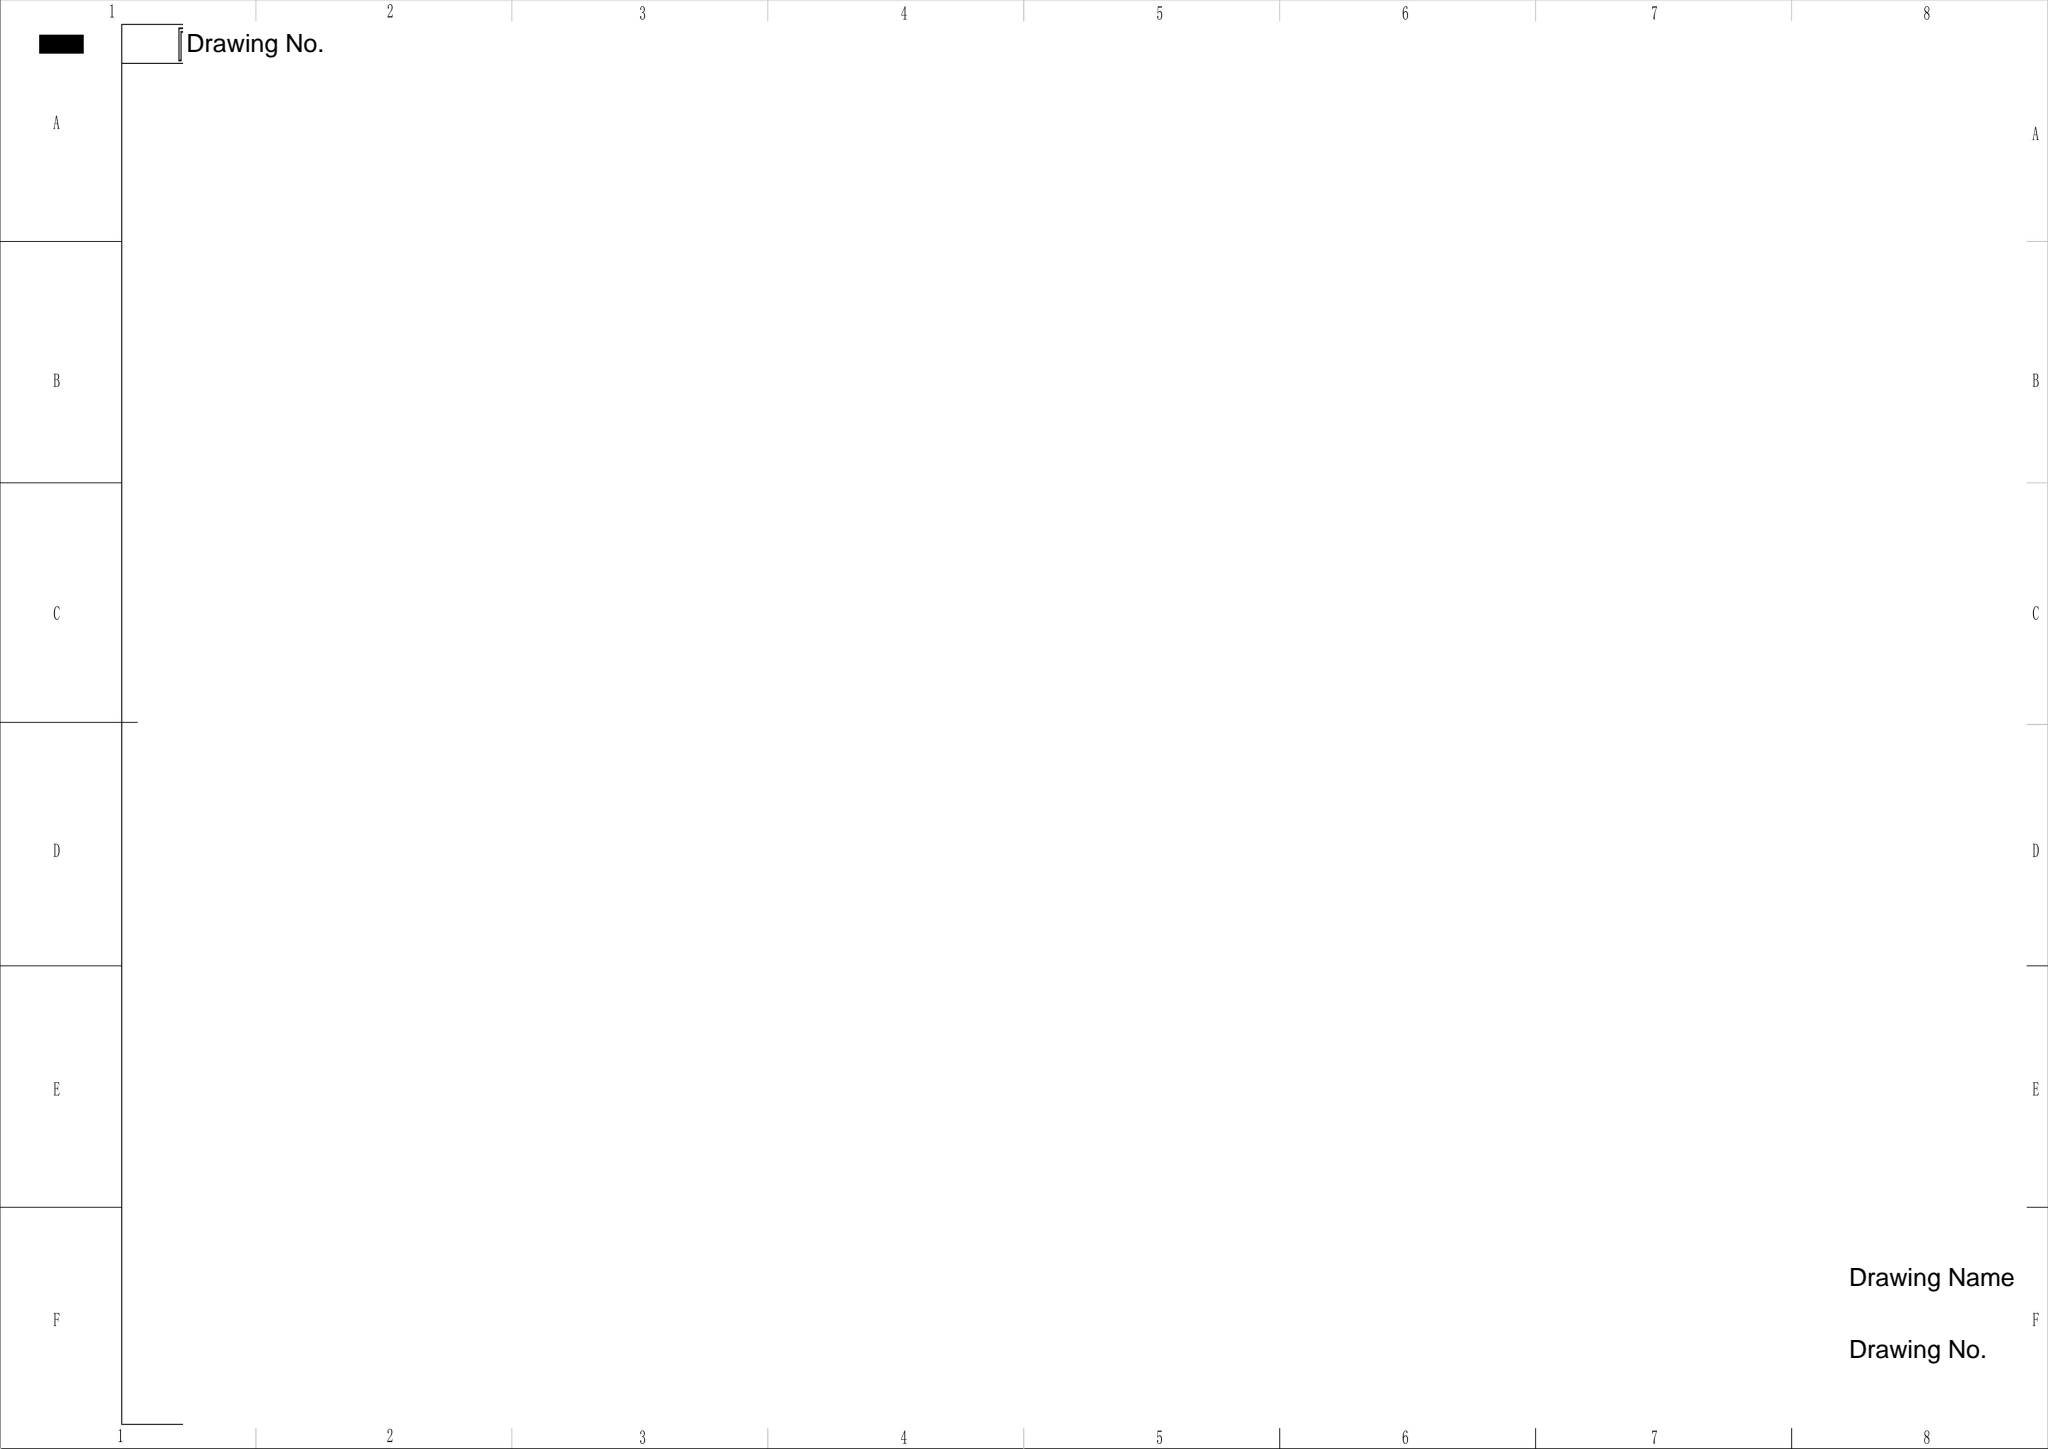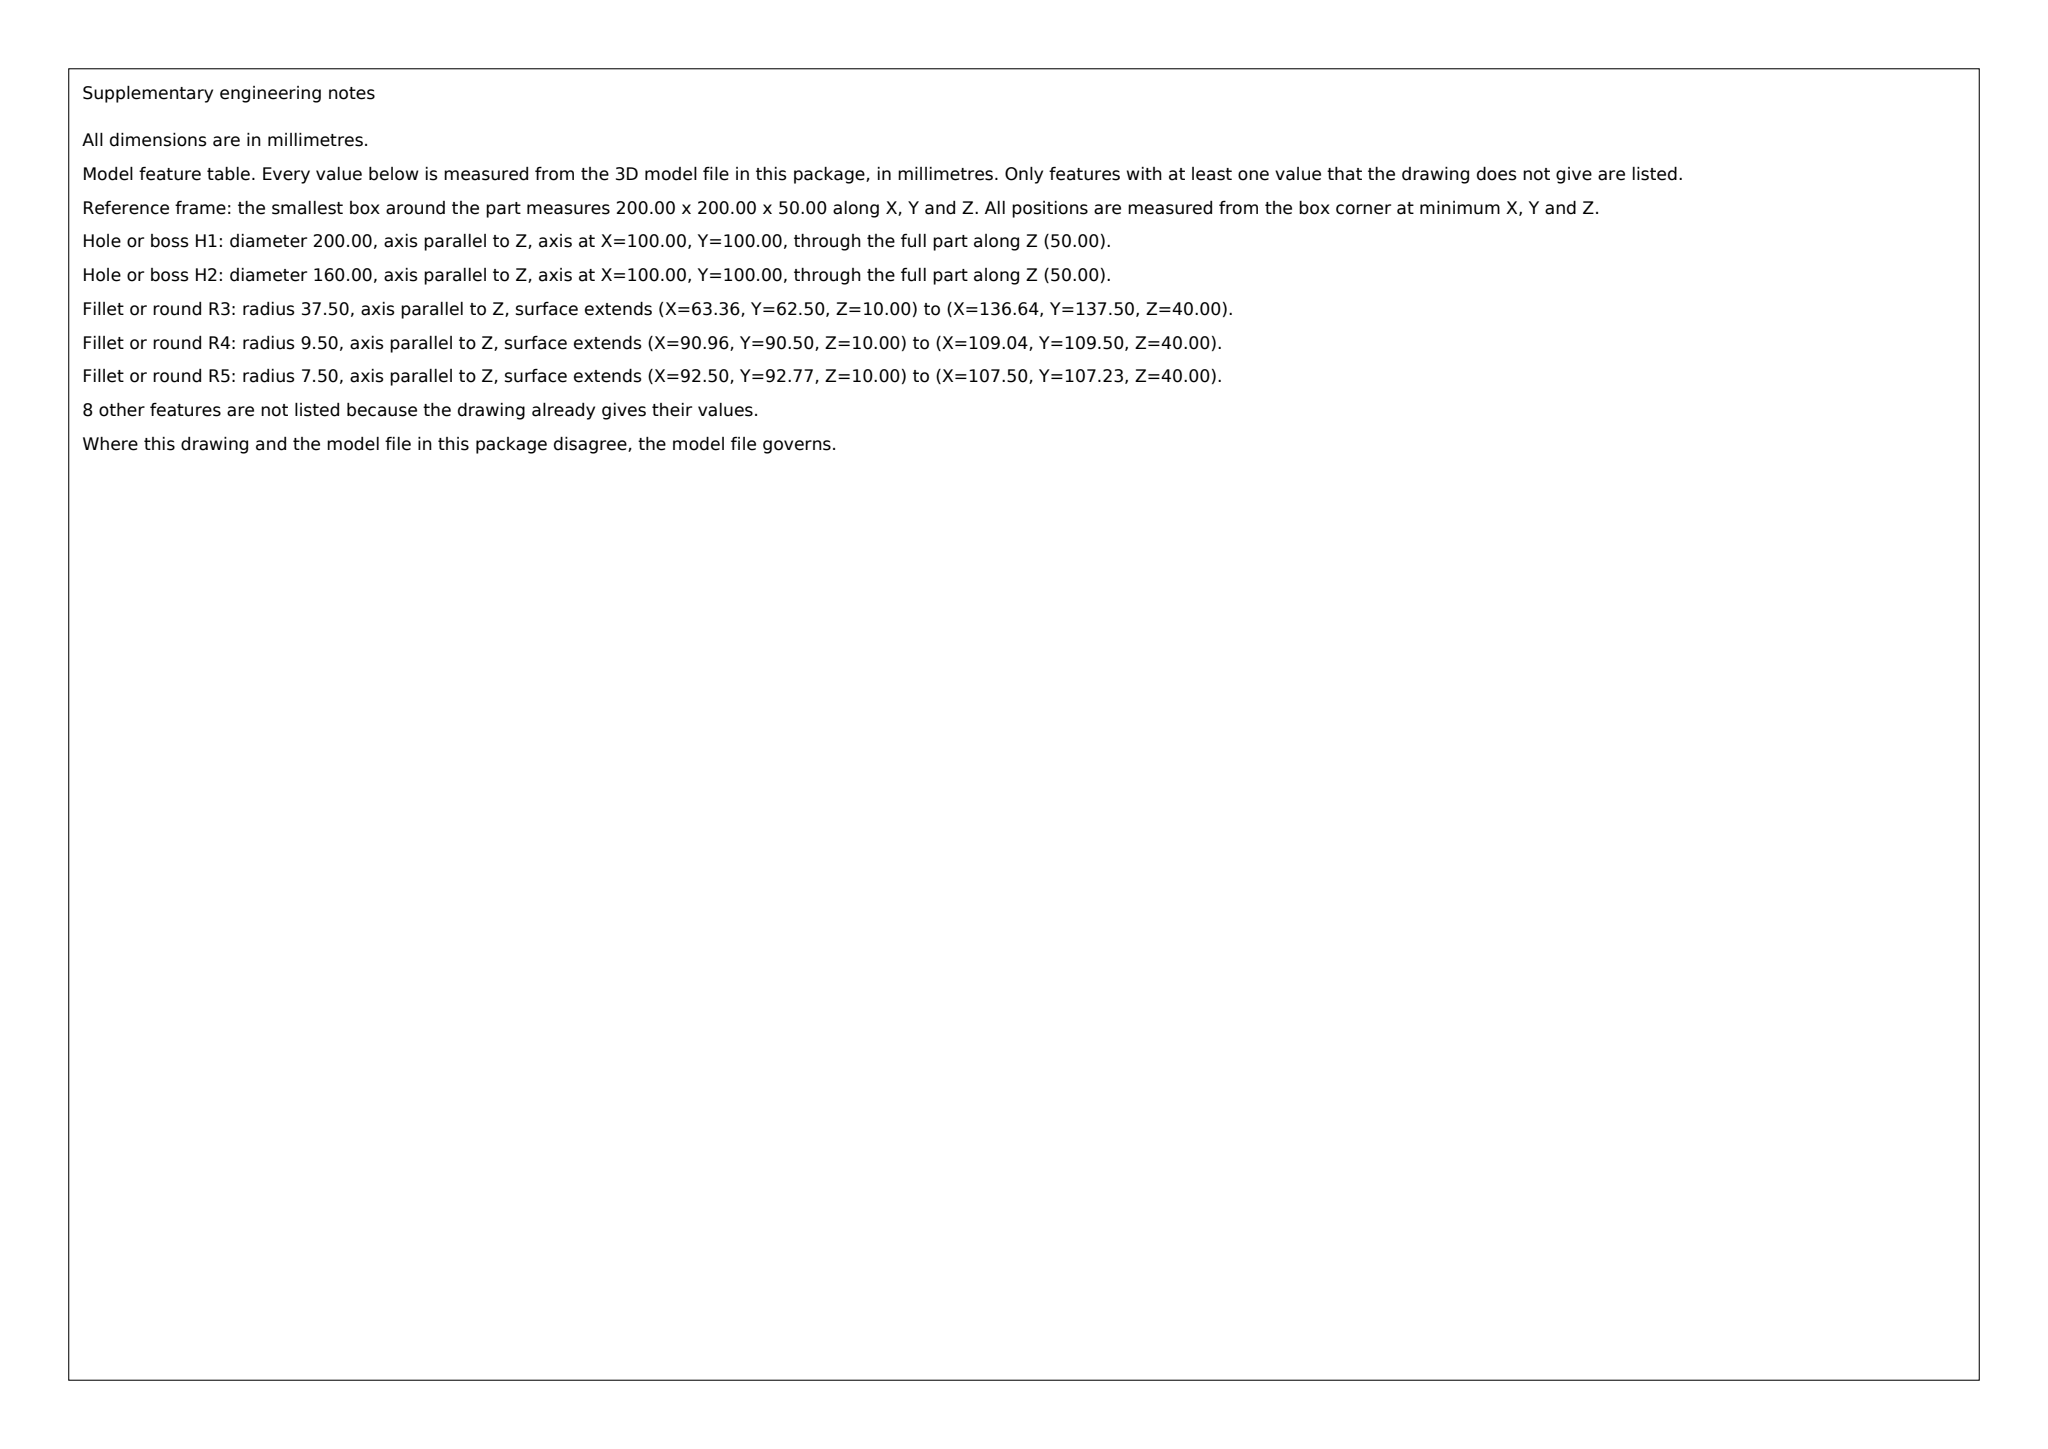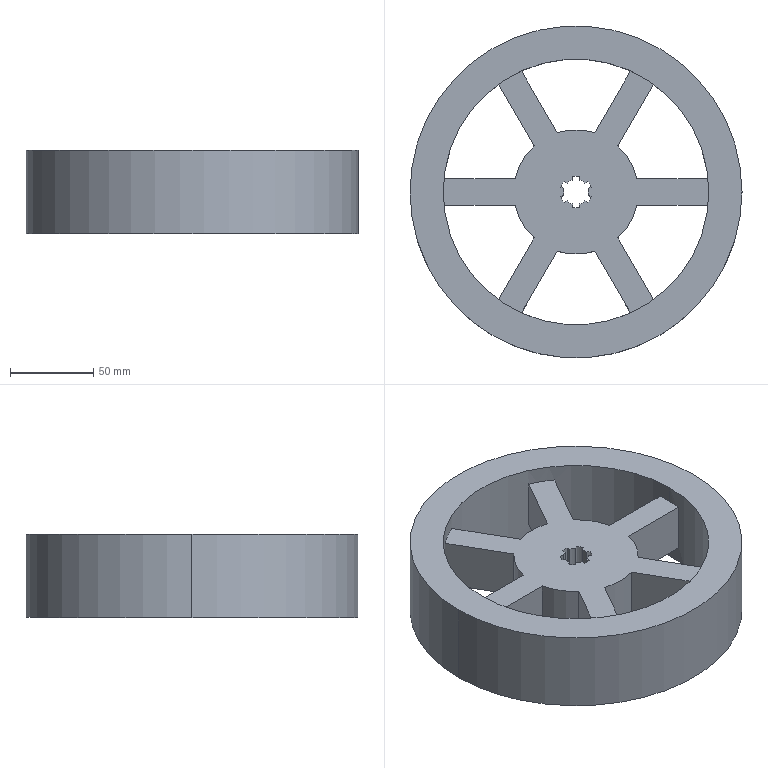Part | SolidWorks | mm | 1 solid | 51 faces | box 200 x 200 x 50 mm | volume 814108 mm3 | plane 28 | cylinder 23 | commonest cylinder face diameters 15 x7 75 x6 19 x6 160 x2 200 x2
build123d program:
from build123d import *

# Parameters (mm, degrees)
SKETCH1_R           = 100
BOSS_EXTRUDE1_DEPTH = 25
SKETCH2_R           = 80
CUT_EXTRUDE1_DEPTH  = 10
CUT_EXTRUDE3_DEPTH  = 147.969
CUT_EXTRUDE4_DEPTH  = 147.969


with BuildPart() as part:
    # Sketch1 → Boss-Extrude1 (new, symmetric)
    with BuildSketch(Plane.XY):
        Circle(SKETCH1_R)
    extrude(amount=BOSS_EXTRUDE1_DEPTH, both=True)

    # Sketch2 → Cut-Extrude1 (cut)
    with BuildSketch(Plane.XY.offset(25)):
        Circle(SKETCH2_R)
    cut_extrude1 = extrude(amount=-CUT_EXTRUDE1_DEPTH, mode=Mode.SUBTRACT)

    # Mirror1: Cut-Extrude1 across plane
    add(cut_extrude1.mirror(Plane.XY), mode=Mode.SUBTRACT)

    # Sketch3 → Cut-Extrude3 (cut, through all)
    with BuildSketch(Plane.XY.offset(15)):
        with BuildLine():
            ThreePointArc((-36.637, 8), (-32.476, 18.75), (-25.247, 27.728))
            Line((-25.247, 27.728), (-46.728, 64.935))
            ThreePointArc((-46.728, 64.935), (-69.282, 40), (-79.599, 8))
            Line((-79.599, 8), (-36.637, 8))
        make_face()
        with BuildLine():
            ThreePointArc((32.871, 72.935), (0, 80), (-32.871, 72.935))
            Line((-32.871, 72.935), (-11.39, 35.728))
            ThreePointArc((-11.39, 35.728), (0, 37.5), (11.39, 35.728))
            Line((11.39, 35.728), (32.871, 72.935))
        make_face()
        with BuildLine():
            ThreePointArc((79.599, 8), (69.282, 40), (46.728, 64.935))
            Line((46.728, 64.935), (25.247, 27.728))
            ThreePointArc((25.247, 27.728), (32.476, 18.75), (36.637, 8))
            Line((36.637, 8), (79.599, 8))
        make_face()
        with BuildLine():
            Line((25.247, -27.728), (46.728, -64.935))
            ThreePointArc((46.728, -64.935), (69.282, -40), (79.599, -8))
            Line((79.599, -8), (36.637, -8))
            ThreePointArc((36.637, -8), (32.476, -18.75), (25.247, -27.728))
        make_face()
        with BuildLine():
            Line((-11.39, -35.728), (-32.871, -72.935))
            ThreePointArc((-32.871, -72.935), (0, -80), (32.871, -72.935))
            Line((32.871, -72.935), (11.39, -35.728))
            ThreePointArc((11.39, -35.728), (0, -37.5), (-11.39, -35.728))
        make_face()
        with BuildLine():
            Line((-36.637, -8), (-79.599, -8))
            ThreePointArc((-79.599, -8), (-69.282, -40), (-46.728, -64.935))
            Line((-46.728, -64.935), (-25.247, -27.728))
            ThreePointArc((-25.247, -27.728), (-32.476, -18.75), (-36.637, -8))
        make_face()
    extrude(amount=-CUT_EXTRUDE3_DEPTH, mode=Mode.SUBTRACT)

    # Sketch4 → Cut-Extrude4 (cut, through all)
    with BuildSketch(Plane(origin=(0, 0, -15), x_dir=(-1, 0, 0), z_dir=(0, 0, -1))):
        with BuildLine():
            Line((-2, 9.287), (-2, 7.228))
            ThreePointArc((-2, 7.228), (-3.75, 6.495), (-5.26, 5.346))
            Line((-5.26, 5.346), (-7.043, 6.376))
            ThreePointArc((-7.043, 6.376), (-8.227, 4.75), (-9.043, 2.911))
            Line((-9.043, 2.911), (-7.26, 1.882))
            ThreePointArc((-7.26, 1.882), (-7.5, 0), (-7.26, -1.882))
            Line((-7.26, -1.882), (-9.043, -2.911))
            ThreePointArc((-9.043, -2.911), (-8.227, -4.75), (-7.043, -6.376))
            Line((-7.043, -6.376), (-5.26, -5.346))
            ThreePointArc((-5.26, -5.346), (-3.75, -6.495), (-2, -7.228))
            Line((-2, -7.228), (-2, -9.287))
            ThreePointArc((-2, -9.287), (0, -9.5), (2, -9.287))
            Line((2, -9.287), (2, -7.228))
            ThreePointArc((2, -7.228), (3.75, -6.495), (5.26, -5.346))
            Line((5.26, -5.346), (7.043, -6.376))
            ThreePointArc((7.043, -6.376), (8.227, -4.75), (9.043, -2.911))
            Line((9.043, -2.911), (7.26, -1.882))
            ThreePointArc((7.26, -1.882), (7.5, 0), (7.26, 1.882))
            Line((7.26, 1.882), (9.043, 2.911))
            ThreePointArc((9.043, 2.911), (8.227, 4.75), (7.043, 6.376))
            Line((7.043, 6.376), (5.26, 5.346))
            ThreePointArc((5.26, 5.346), (3.75, 6.495), (2, 7.228))
            Line((2, 7.228), (2, 9.287))
            ThreePointArc((2, 9.287), (0, 9.5), (-2, 9.287))
        make_face()
    extrude(amount=-CUT_EXTRUDE4_DEPTH, mode=Mode.SUBTRACT)


solid = part.part